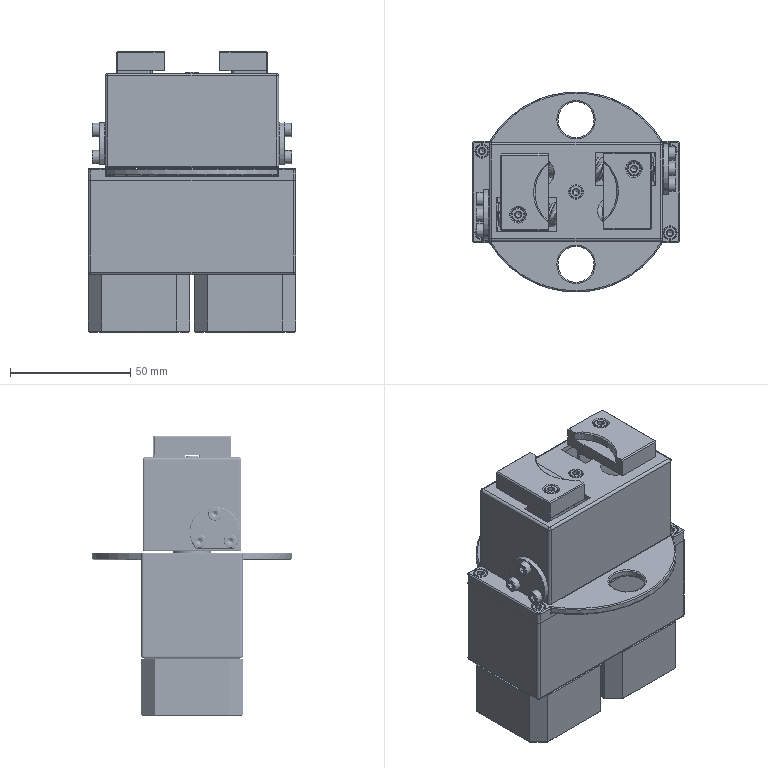Assembly | NX | mm | 51 component files | 54 solids | 2276 faces | box 86 x 83 x 116.5 mm | volume 198623 mm3 | plane 738 | cylinder 526 | other 395 | cone 379 | spline 141 | torus 69 | sphere 28 | commonest cylinder face diameters 1 x94 2 x40 11 x37 7.125 x36 8.4 x32 24.5 x27 10 x26 5.5 x25
Bill of materials:
unnamed part 1 | 2 |  | Square prismatic body with chamfered vertical corners. One face has a shallow circular raised boss and a single cylindrical shaft sticking out from the center. Small holes sit near the four corners of the face.
unnamed part 2 | 1 |  | Short thick cylindrical ring with a central through bore and a larger counterbore on one face. Outer edges are chamfered.
unnamed part 3 | 1 |  | Long straight thin-walled cylindrical tube with plain square-cut ends.
unnamed part 4 | 1 |  | Open-top rectangular box housing with a flat rim carrying corner holes. The floor has two large round openings, a central raised ring boss with a small bore, four smaller holes, and internal wall notches.
unnamed part 5 | 2 |  | Solid straight cylindrical rod with small edge chamfers at both ends.
unnamed part 6 | 2 |  | Combined gear element: a helical worm thread section runs along most of the length, with an integral spur pinion at one end and a central through bore.
unnamed part 7 | 1 |  | Hollow cylindrical part with toothed sections at both ends, a smooth larger-diameter plain band in the middle, and short plain journals at the extreme ends.
unnamed part 8 | 1 |  | Worm-type cylinder with a single helical thread over most of its length. A plain cylindrical collar sits at one end, and a small stepped boss with a central bore is at the other end.
unnamed part 9 | 1 |  | Short solid cylindrical pin with chamfered ends.
unnamed part 10 | 2 |  | Rectangular block with a raised tongue or rib on the top face holding a small hole. A face has two rounded-rectangle through windows and a lower round hole with irregular lobed internal geometry. The bottom corners are chamfered.
unnamed part 11 | 1 |  | Long slender hollow tube or shaft with a central bore. A local flat or reduced section runs along part of its length, with a short angled cut or notch near one end.
unnamed part 12 | 2 |  | Flanged part: a circular flange truncated by a straight flat edge, carrying three through holes, with a projecting cylindrical boss that has a central hole.
unnamed part 13 | 25 |  | Socket-head-cap-screw-like shape: a cylindrical head with a rounded top edge and a hexagonal socket recess, on a plain smaller-diameter cylindrical shank.
unnamed part 14 | 1 |  | Small spur gear (pinion) with a cylindrical hub on one side. It has a D-shaped bore through the center and one radial hole through the hub wall.
unnamed part 15 | 1 |  | Thin spur gear with a short hub boss on one face, a D-shaped center bore, and six round lightening holes evenly spaced around the bore.
unnamed part 16 | 2 |  | Solid cylindrical pin or rod with chamfered edges at both ends and flat end faces.
unnamed part 17 | 1 |  | Rectangular block or housing with slightly rounded edges. The top face has two rectangular openings, two larger round holes and one small center hole. One end face has a circular recess or boss outline with three small holes around it. A short cylindrical protrusion sticks out of one side.
unnamed part 18 | 2 |  | Rectangular block with chamfered edges, one counterbored through-hole near one corner, and a curved, arc-shaped stepped cut-out along one long edge of the top face.
unnamed part 19 | 1 |  | Hollow cylindrical tube with an evenly spaced series of circumferential ribs or grooves along its whole length and a plain through-bore.
unnamed part 20 | 1 |  | Mostly circular flat plate with two opposite rectangular tab extensions. It has a central counterbored hole, two large round holes, two medium holes, several small mounting holes in the tabs, and downward lugs, one of which has a hole.
Mates:
1. fix | assembly component
2. bond | GB70_2-M3x6 17 component | assembly component
3. bond | GB70_2-M3x6 16 component | assembly component
4. bond | GB70_2-M3x6 15 component | assembly component
5. circular | assembly datumaxis | assembly cartesiancoordinatesystem | assembly cartesiancoordinatesystem | assembly cartesiancoordinatesystem
6. fix | assembly component
7. bond | DJZ_11_threaded_shaft_LH 2 component | assembly component
8. bond | GB120-3x45 2 component | assembly component
9. bond | GB70_2-M3x6 17 component | assembly component
10. bond | DJZ_09_end_cap 2 component | assembly component
11. bond | GB70_2-M3x6 16 component | assembly component
12. bond | DJZ_12_jaw_nut_LH 2 component | assembly component
13. bond | GB70_2-M3x6 15 component | assembly component
14. bond | DJZ_11_threaded_shaft_LH 1 component | assembly component
15. bond | GB120-3x45 1 component | assembly component
16. bond | GB70_2-M3x6 14 component | assembly component
17. bond | DJZ_09_end_cap 1 component | assembly component
18. bond | GB70_2-M3x6 13 component | assembly component
19. bond | DJZ_12_jaw_nut_LH 1 component | assembly component
20. bond | GB70_2-M3x6 12 component | assembly component
21. circular | assembly datumaxis | assembly cartesiancoordinatesystem | assembly cartesiancoordinatesystem
22. circular | assembly datumaxis | assembly cartesiancoordinatesystem | assembly cartesiancoordinatesystem
23. circular | assembly datumaxis | assembly cartesiancoordinatesystem | assembly cartesiancoordinatesystem
24. circular | assembly datumaxis | assembly cartesiancoordinatesystem | assembly cartesiancoordinatesystem
25. circular | assembly datumaxis | assembly cartesiancoordinatesystem | assembly cartesiancoordinatesystem
26. circular | assembly datumaxis | assembly cartesiancoordinatesystem | assembly cartesiancoordinatesystem
27. circular | assembly datumaxis | assembly cartesiancoordinatesystem | assembly cartesiancoordinatesystem
28. concentric | DJZ_13_jaw 2 edge | DJZ_12_jaw_nut_LH 2 edge
29. concentric | GB70_2-M3x6 2 edge | DJZ_13_jaw 2 edge
30. fix | assembly component
31. bond | DJZ_13_jaw 2 component | assembly component
32. bond | GB70_2-M3x6 2 component | assembly component
33. bond | DJZ_13_jaw 1 component | assembly component
34. bond | GB70_2-M3x6 1 component | assembly component
35. circular | assembly datumaxis | assembly cartesiancoordinatesystem | assembly cartesiancoordinatesystem
36. circular | assembly datumaxis | assembly cartesiancoordinatesystem | assembly cartesiancoordinatesystem